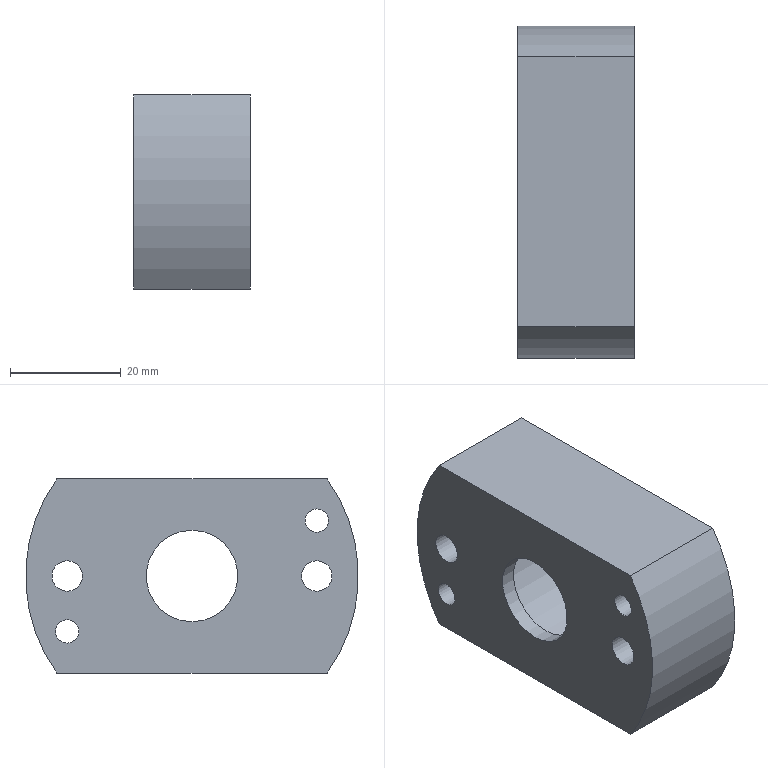Component | NX | SLIDE_BEARING_BLOCK | 1 solid | 19 faces | volume 26049 mm3 | cylinder 11 | plane 8 | commonest cylinder face diameters 60 x2 5.5 x2 9 x2 4.2 x2 16.5 x1 30 x1 20 x1